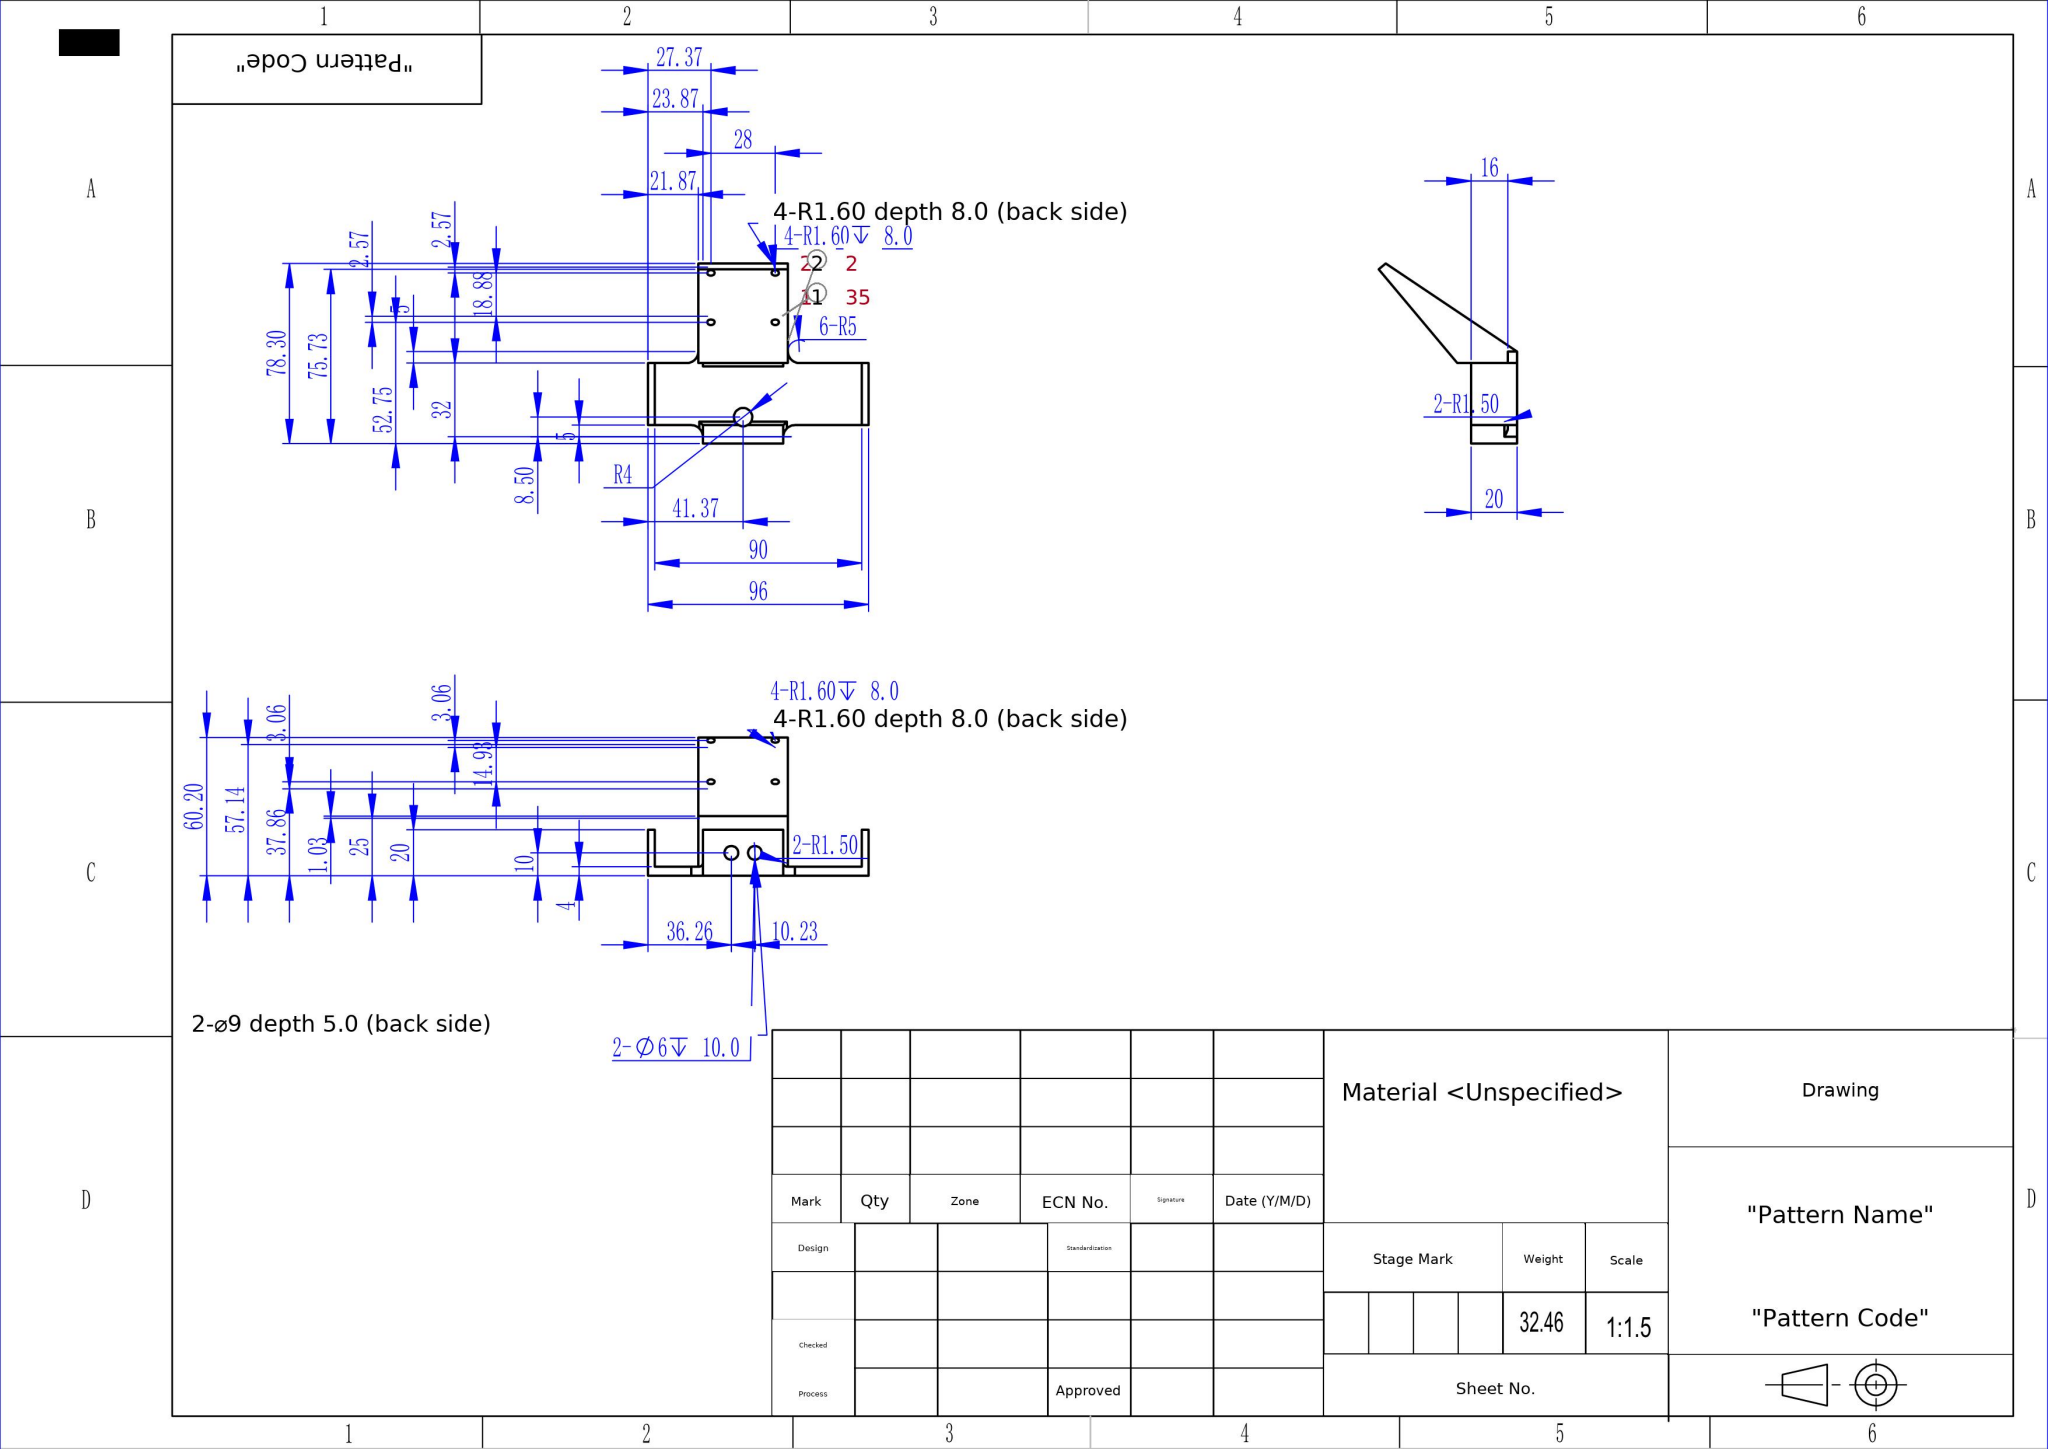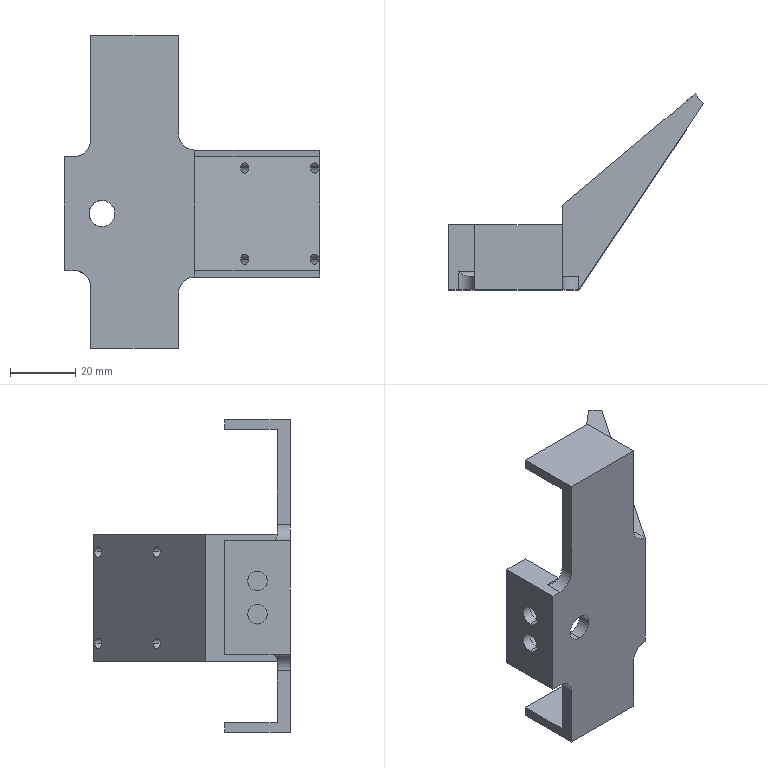Part | SolidWorks | mm | material <Unspecified> | 1 solid | 62 faces | box 78.3 x 60.2 x 96 mm | volume 32465 mm3 | plane 35 | cylinder 27 | commonest cylinder face diameters 3.2 x8 3 x5 6 x4 9 x4 10 x4 8 x2